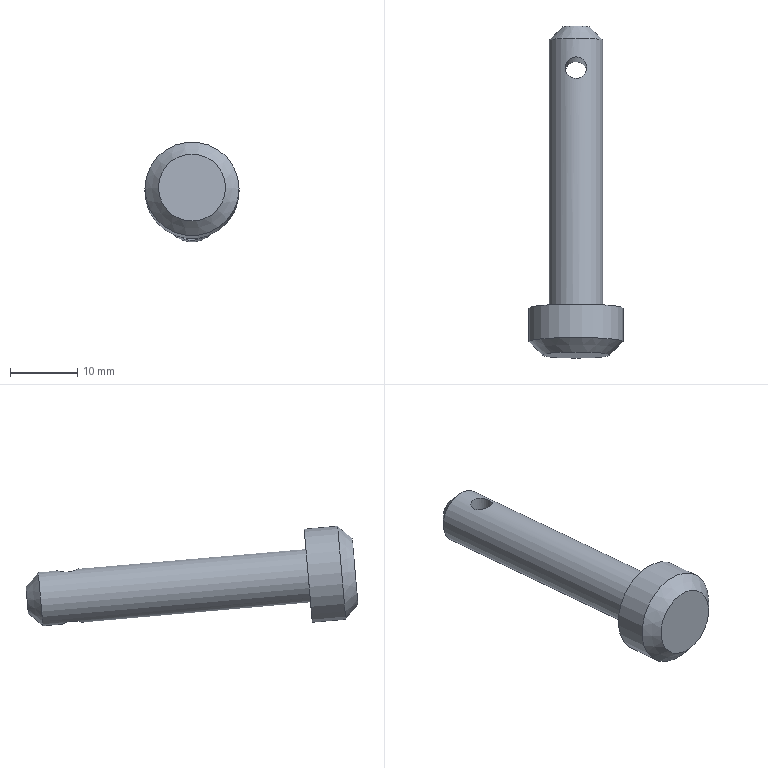Component | NX | PIN | 1 solid | 8 faces | box 14 x 49.42 x 14.88 mm | volume 3004 mm3 | cylinder 3 | plane 3 | cone 2 | commonest cylinder face diameters 8 x1 14 x1 3.2 x1
STEP:
#1=CARTESIAN_POINT('',(0.,0.,0.));
#2=DIRECTION('',(0.,0.,1.));
#3=DIRECTION('',(1.,0.,0.));
#4=AXIS2_PLACEMENT_3D('',#1,#2,#3);
#5=CARTESIAN_POINT('',(279.941,470.083,-25.853));
#6=VERTEX_POINT('',#5);
#7=CARTESIAN_POINT('',(275.941,470.083,-25.853));
#8=DIRECTION('',(0.,-0.9962,0.08716));
#9=DIRECTION('',(1.,0.,0.));
#10=AXIS2_PLACEMENT_3D('',#7,#8,#9);
#11=CIRCLE('',#10,4.);
#12=CARTESIAN_POINT('',(275.941,430.235,-22.367));
#13=DIRECTION('',(0.,0.9962,-0.08716));
#14=DIRECTION('',(-1.,0.,0.));
#15=AXIS2_PLACEMENT_3D('',#12,#13,#14);
#16=CYLINDRICAL_SURFACE('',#15,4.);
#17=CARTESIAN_POINT('',(9.425,40.));
#18=DIRECTION('',(-1.,0.));
#19=VECTOR('',#18,1.);
#20=LINE('',#17,#19);
#21=(GEOMETRIC_REPRESENTATION_CONTEXT(2)PARAMETRIC_REPRESENTATION_CONTEXT()REPRESENTATION_CONTEXT('',''));
#22=DEFINITIONAL_REPRESENTATION('',(#20),#21);
#23=PCURVE('',#16,#22);
#24=CARTESIAN_POINT('',(275.941,470.083,-25.853));
#25=DIRECTION('',(0.,-0.9962,0.08716));
#26=DIRECTION('',(1.,-0.,-0.));
#27=AXIS2_PLACEMENT_3D('',#24,#25,#26);
#28=CONICAL_SURFACE('',#27,4.,0.7854);
#29=CARTESIAN_POINT('',(0.,0.));
#30=DIRECTION('',(1.,0.));
#31=VECTOR('',#30,1.);
#32=LINE('',#29,#31);
#33=(GEOMETRIC_REPRESENTATION_CONTEXT(2)PARAMETRIC_REPRESENTATION_CONTEXT()REPRESENTATION_CONTEXT('',''));
#34=DEFINITIONAL_REPRESENTATION('',(#32),#33);
#35=PCURVE('',#28,#34);
#36=SURFACE_CURVE('',#11,(#23,#35),.PCURVE_S1.);
#37=EDGE_CURVE('',#6,#6,#36,.T.);
#38=ORIENTED_EDGE('',*,*,#37,.T.);
#39=CARTESIAN_POINT('',(279.941,430.235,-22.367));
#40=VERTEX_POINT('',#39);
#41=CARTESIAN_POINT('',(279.941,430.235,-22.367));
#42=CARTESIAN_POINT('',(279.941,470.083,-25.853));
#43=B_SPLINE_CURVE_WITH_KNOTS('',1,(#41,#42),.UNSPECIFIED.,.F.,.F.,(2,2),(0.,40.),.PIECEWISE_BEZIER_KNOTS.);
#44=CARTESIAN_POINT('',(3.142,0.));
#45=DIRECTION('',(0.,1.));
#46=VECTOR('',#45,1.);
#47=LINE('',#44,#46);
#48=(GEOMETRIC_REPRESENTATION_CONTEXT(2)PARAMETRIC_REPRESENTATION_CONTEXT()REPRESENTATION_CONTEXT('',''));
#49=DEFINITIONAL_REPRESENTATION('',(#47),#48);
#50=PCURVE('',#16,#49);
#51=CARTESIAN_POINT('',(9.425,0.));
#52=DIRECTION('',(0.,1.));
#53=VECTOR('',#52,1.);
#54=LINE('',#51,#53);
#55=(GEOMETRIC_REPRESENTATION_CONTEXT(2)PARAMETRIC_REPRESENTATION_CONTEXT()REPRESENTATION_CONTEXT('',''));
#56=DEFINITIONAL_REPRESENTATION('',(#54),#55);
#57=PCURVE('',#16,#56);
#58=SEAM_CURVE('',#43,(#50,#57),.PCURVE_S1.);
#59=EDGE_CURVE('',#40,#6,#58,.T.);
#60=ORIENTED_EDGE('',*,*,#59,.F.);
#61=CARTESIAN_POINT('',(275.941,430.235,-22.367));
#62=DIRECTION('',(0.,-0.9962,0.08716));
#63=DIRECTION('',(1.,0.,0.));
#64=AXIS2_PLACEMENT_3D('',#61,#62,#63);
#65=CIRCLE('',#64,4.);
#66=CARTESIAN_POINT('',(9.425,0.));
#67=DIRECTION('',(-1.,0.));
#68=VECTOR('',#67,1.);
#69=LINE('',#66,#68);
#70=(GEOMETRIC_REPRESENTATION_CONTEXT(2)PARAMETRIC_REPRESENTATION_CONTEXT()REPRESENTATION_CONTEXT('',''));
#71=DEFINITIONAL_REPRESENTATION('',(#69),#70);
#72=PCURVE('',#16,#71);
#73=CARTESIAN_POINT('',(275.941,430.235,-22.367));
#74=DIRECTION('',(0.,-0.9962,0.08716));
#75=DIRECTION('',(1.,0.,0.));
#76=AXIS2_PLACEMENT_3D('',#73,#74,#75);
#77=PLANE('',#76);
#78=CARTESIAN_POINT('',(0.,0.));
#79=DIRECTION('',(1.,0.));
#80=AXIS2_PLACEMENT_2D('',#78,#79);
#81=CIRCLE('',#80,4.);
#82=(GEOMETRIC_REPRESENTATION_CONTEXT(2)PARAMETRIC_REPRESENTATION_CONTEXT()REPRESENTATION_CONTEXT('',''));
#83=DEFINITIONAL_REPRESENTATION('',(#81),#82);
#84=PCURVE('',#77,#83);
#85=SURFACE_CURVE('',#65,(#72,#84),.PCURVE_S1.);
#86=EDGE_CURVE('',#40,#40,#85,.T.);
#87=ORIENTED_EDGE('',*,*,#86,.F.);
#88=ORIENTED_EDGE('',*,*,#59,.T.);
#89=EDGE_LOOP('',(#38,#60,#87,#88));
#90=FACE_BOUND('',#89,.T.);
#91=CARTESIAN_POINT('',(275.941,464.455,-21.345));
#92=VERTEX_POINT('',#91);
#93=CARTESIAN_POINT('',(275.941,464.455,-21.345));
#94=CARTESIAN_POINT('',(276.113,464.455,-21.345));
#95=CARTESIAN_POINT('',(276.287,464.482,-21.359));
#96=CARTESIAN_POINT('',(276.448,464.534,-21.384));
#97=CARTESIAN_POINT('',(276.609,464.586,-21.41));
#98=CARTESIAN_POINT('',(276.763,464.663,-21.446));
#99=CARTESIAN_POINT('',(276.897,464.761,-21.488));
#100=CARTESIAN_POINT('',(277.038,464.862,-21.532));
#101=CARTESIAN_POINT('',(277.162,464.987,-21.582));
#102=CARTESIAN_POINT('',(277.261,465.128,-21.629));
#103=CARTESIAN_POINT('',(277.364,465.275,-21.678));
#104=CARTESIAN_POINT('',(277.443,465.444,-21.725));
#105=CARTESIAN_POINT('',(277.49,465.621,-21.76));
#106=CARTESIAN_POINT('',(277.534,465.79,-21.794));
#107=CARTESIAN_POINT('',(277.55,465.972,-21.817));
#108=CARTESIAN_POINT('',(277.536,466.149,-21.826));
#109=CARTESIAN_POINT('',(277.522,466.314,-21.835));
#110=CARTESIAN_POINT('',(277.483,466.479,-21.832));
#111=CARTESIAN_POINT('',(277.42,466.632,-21.82));
#112=CARTESIAN_POINT('',(277.356,466.788,-21.808));
#113=CARTESIAN_POINT('',(277.268,466.935,-21.788));
#114=CARTESIAN_POINT('',(277.16,467.064,-21.764));
#115=CARTESIAN_POINT('',(277.045,467.203,-21.739));
#116=CARTESIAN_POINT('',(276.905,467.323,-21.711));
#117=CARTESIAN_POINT('',(276.75,467.417,-21.687));
#118=CARTESIAN_POINT('',(276.592,467.511,-21.663));
#119=CARTESIAN_POINT('',(276.415,467.58,-21.642));
#120=CARTESIAN_POINT('',(276.233,467.615,-21.632));
#121=CARTESIAN_POINT('',(276.061,467.648,-21.622));
#122=CARTESIAN_POINT('',(275.882,467.651,-21.621));
#123=CARTESIAN_POINT('',(275.709,467.625,-21.629));
#124=CARTESIAN_POINT('',(275.544,467.6,-21.637));
#125=CARTESIAN_POINT('',(275.382,467.548,-21.652));
#126=CARTESIAN_POINT('',(275.234,467.473,-21.672));
#127=CARTESIAN_POINT('',(275.082,467.396,-21.693));
#128=CARTESIAN_POINT('',(274.941,467.293,-21.719));
#129=CARTESIAN_POINT('',(274.821,467.173,-21.743));
#130=CARTESIAN_POINT('',(274.693,467.044,-21.77));
#131=CARTESIAN_POINT('',(274.585,466.892,-21.795));
#132=CARTESIAN_POINT('',(274.505,466.728,-21.812));
#133=CARTESIAN_POINT('',(274.425,466.562,-21.828));
#134=CARTESIAN_POINT('',(274.371,466.379,-21.836));
#135=CARTESIAN_POINT('',(274.351,466.195,-21.828));
#136=CARTESIAN_POINT('',(274.332,466.025,-21.822));
#137=CARTESIAN_POINT('',(274.341,465.849,-21.802));
#138=CARTESIAN_POINT('',(274.377,465.684,-21.772));
#139=CARTESIAN_POINT('',(274.412,465.525,-21.744));
#140=CARTESIAN_POINT('',(274.472,465.372,-21.705));
#141=CARTESIAN_POINT('',(274.553,465.235,-21.663));
#142=CARTESIAN_POINT('',(274.638,465.089,-21.618));
#143=CARTESIAN_POINT('',(274.748,464.957,-21.569));
#144=CARTESIAN_POINT('',(274.876,464.847,-21.524));
#145=CARTESIAN_POINT('',(275.011,464.729,-21.476));
#146=CARTESIAN_POINT('',(275.171,464.633,-21.432));
#147=CARTESIAN_POINT('',(275.341,464.567,-21.4));
#148=CARTESIAN_POINT('',(275.508,464.502,-21.369));
#149=CARTESIAN_POINT('',(275.691,464.464,-21.349));
#150=CARTESIAN_POINT('',(275.873,464.456,-21.346));
#151=CARTESIAN_POINT('',(275.896,464.455,-21.345));
#152=CARTESIAN_POINT('',(275.918,464.455,-21.345));
#153=CARTESIAN_POINT('',(275.941,464.455,-21.345));
#154=B_SPLINE_CURVE_WITH_KNOTS('',3,(#93,#94,#95,#96,#97,#98,#99,#100,#101,#102,#103,#104,#105,#106,#107,#108,#109,#110,#111,#112,#113,#114,#115,#116,#117,#118,#119,#120,#121,#122,#123,#124,#125,#126,#127,#128,#129,#130,#131,#132,#133,#134,#135,#136,#137,#138,#139,#140,#141,#142,#143,#144,#145,#146,#147,#148,#149,#150,#151,#152,#153),.UNSPECIFIED.,.T.,.F.,(1,3,3,3,3,3,3,3,3,3,3,3,3,3,3,3,3,3,3,3,3,3,1),(-0.006652,0.,0.05091,0.1017,0.1546,0.2101,0.2629,0.312,0.3621,0.4161,0.4713,0.5231,0.5725,0.6234,0.6778,0.7328,0.7837,0.8325,0.8842,0.9393,0.9933,1.,1.051),.UNSPECIFIED.);
#155=CARTESIAN_POINT('',(7.854,34.));
#156=CARTESIAN_POINT('',(7.864,34.));
#157=CARTESIAN_POINT('',(7.883,34.003));
#158=CARTESIAN_POINT('',(7.912,34.015));
#159=CARTESIAN_POINT('',(7.94,34.036));
#160=CARTESIAN_POINT('',(7.968,34.065));
#161=CARTESIAN_POINT('',(7.995,34.101));
#162=CARTESIAN_POINT('',(8.022,34.145));
#163=CARTESIAN_POINT('',(8.048,34.197));
#164=CARTESIAN_POINT('',(8.073,34.255));
#165=CARTESIAN_POINT('',(8.097,34.32));
#166=CARTESIAN_POINT('',(8.119,34.391));
#167=CARTESIAN_POINT('',(8.141,34.468));
#168=CARTESIAN_POINT('',(8.161,34.551));
#169=CARTESIAN_POINT('',(8.18,34.639));
#170=CARTESIAN_POINT('',(8.197,34.732));
#171=CARTESIAN_POINT('',(8.212,34.829));
#172=CARTESIAN_POINT('',(8.226,34.931));
#173=CARTESIAN_POINT('',(8.238,35.036));
#174=CARTESIAN_POINT('',(8.248,35.145));
#175=CARTESIAN_POINT('',(8.256,35.255));
#176=CARTESIAN_POINT('',(8.261,35.369));
#177=CARTESIAN_POINT('',(8.265,35.484));
#178=CARTESIAN_POINT('',(8.266,35.599));
#179=CARTESIAN_POINT('',(8.265,35.714));
#180=CARTESIAN_POINT('',(8.261,35.829));
#181=CARTESIAN_POINT('',(8.256,35.942));
#182=CARTESIAN_POINT('',(8.248,36.054));
#183=CARTESIAN_POINT('',(8.238,36.163));
#184=CARTESIAN_POINT('',(8.226,36.268));
#185=CARTESIAN_POINT('',(8.213,36.37));
#186=CARTESIAN_POINT('',(8.197,36.467));
#187=CARTESIAN_POINT('',(8.18,36.561));
#188=CARTESIAN_POINT('',(8.161,36.649));
#189=CARTESIAN_POINT('',(8.141,36.731));
#190=CARTESIAN_POINT('',(8.12,36.809));
#191=CARTESIAN_POINT('',(8.097,36.88));
#192=CARTESIAN_POINT('',(8.073,36.945));
#193=CARTESIAN_POINT('',(8.048,37.003));
#194=CARTESIAN_POINT('',(8.022,37.054));
#195=CARTESIAN_POINT('',(7.996,37.098));
#196=CARTESIAN_POINT('',(7.968,37.135));
#197=CARTESIAN_POINT('',(7.94,37.164));
#198=CARTESIAN_POINT('',(7.912,37.184));
#199=CARTESIAN_POINT('',(7.883,37.197));
#200=CARTESIAN_POINT('',(7.854,37.201));
#201=CARTESIAN_POINT('',(7.825,37.197));
#202=CARTESIAN_POINT('',(7.797,37.185));
#203=CARTESIAN_POINT('',(7.768,37.164));
#204=CARTESIAN_POINT('',(7.74,37.136));
#205=CARTESIAN_POINT('',(7.713,37.099));
#206=CARTESIAN_POINT('',(7.686,37.055));
#207=CARTESIAN_POINT('',(7.66,37.004));
#208=CARTESIAN_POINT('',(7.635,36.946));
#209=CARTESIAN_POINT('',(7.611,36.881));
#210=CARTESIAN_POINT('',(7.589,36.809));
#211=CARTESIAN_POINT('',(7.567,36.733));
#212=CARTESIAN_POINT('',(7.547,36.65));
#213=CARTESIAN_POINT('',(7.528,36.562));
#214=CARTESIAN_POINT('',(7.511,36.469));
#215=CARTESIAN_POINT('',(7.495,36.371));
#216=CARTESIAN_POINT('',(7.482,36.27));
#217=CARTESIAN_POINT('',(7.47,36.165));
#218=CARTESIAN_POINT('',(7.46,36.056));
#219=CARTESIAN_POINT('',(7.452,35.944));
#220=CARTESIAN_POINT('',(7.447,35.831));
#221=CARTESIAN_POINT('',(7.443,35.717));
#222=CARTESIAN_POINT('',(7.442,35.602));
#223=CARTESIAN_POINT('',(7.443,35.486));
#224=CARTESIAN_POINT('',(7.447,35.371));
#225=CARTESIAN_POINT('',(7.452,35.258));
#226=CARTESIAN_POINT('',(7.46,35.147));
#227=CARTESIAN_POINT('',(7.47,35.038));
#228=CARTESIAN_POINT('',(7.482,34.932));
#229=CARTESIAN_POINT('',(7.495,34.83));
#230=CARTESIAN_POINT('',(7.511,34.733));
#231=CARTESIAN_POINT('',(7.528,34.639));
#232=CARTESIAN_POINT('',(7.547,34.551));
#233=CARTESIAN_POINT('',(7.567,34.468));
#234=CARTESIAN_POINT('',(7.588,34.391));
#235=CARTESIAN_POINT('',(7.611,34.32));
#236=CARTESIAN_POINT('',(7.635,34.255));
#237=CARTESIAN_POINT('',(7.66,34.197));
#238=CARTESIAN_POINT('',(7.686,34.145));
#239=CARTESIAN_POINT('',(7.712,34.101));
#240=CARTESIAN_POINT('',(7.74,34.065));
#241=CARTESIAN_POINT('',(7.768,34.036));
#242=CARTESIAN_POINT('',(7.796,34.015));
#243=CARTESIAN_POINT('',(7.825,34.003));
#244=CARTESIAN_POINT('',(7.844,34.));
#245=CARTESIAN_POINT('',(7.854,34.));
#246=B_SPLINE_CURVE_WITH_KNOTS('',3,(#155,#156,#157,#158,#159,#160,#161,#162,#163,#164,#165,#166,#167,#168,#169,#170,#171,#172,#173,#174,#175,#176,#177,#178,#179,#180,#181,#182,#183,#184,#185,#186,#187,#188,#189,#190,#191,#192,#193,#194,#195,#196,#197,#198,#199,#200,#201,#202,#203,#204,#205,#206,#207,#208,#209,#210,#211,#212,#213,#214,#215,#216,#217,#218,#219,#220,#221,#222,#223,#224,#225,#226,#227,#228,#229,#230,#231,#232,#233,#234,#235,#236,#237,#238,#239,#240,#241,#242,#243,#244,#245),.UNSPECIFIED.,.T.,.F.,(4,1,1,1,1,1,1,1,1,1,1,1,1,1,1,1,1,1,1,1,1,1,1,1,1,1,1,1,1,1,1,1,1,1,1,1,1,1,1,1,1,1,1,1,1,1,1,1,1,1,1,1,1,1,1,1,1,1,1,1,1,1,1,1,1,1,1,1,1,1,1,1,1,1,1,1,1,1,1,1,1,1,1,1,1,1,1,1,4),(0.,0.01136,0.02273,0.03409,0.04545,0.05682,0.06818,0.07955,0.09091,0.1023,0.1136,0.125,0.1364,0.1477,0.1591,0.1705,0.1818,0.1932,0.2045,0.2159,0.2273,0.2386,0.25,0.2614,0.2727,0.2841,0.2955,0.3068,0.3182,0.3295,0.3409,0.3523,0.3636,0.375,0.3864,0.3977,0.4091,0.4205,0.4318,0.4432,0.4545,0.4659,0.4773,0.4886,0.5,0.5114,0.5227,0.5341,0.5455,0.5568,0.5682,0.5795,0.5909,0.6023,0.6136,0.625,0.6364,0.6477,0.6591,0.6705,0.6818,0.6932,0.7045,0.7159,0.7273,0.7386,0.75,0.7614,0.7727,0.7841,0.7955,0.8068,0.8182,0.8295,0.8409,0.8523,0.8636,0.875,0.8864,0.8977,0.9091,0.9205,0.9318,0.9432,0.9545,0.9659,0.9773,0.9886,1.),.QUASI_UNIFORM_KNOTS.);
#247=(GEOMETRIC_REPRESENTATION_CONTEXT(2)PARAMETRIC_REPRESENTATION_CONTEXT()REPRESENTATION_CONTEXT('',''));
#248=DEFINITIONAL_REPRESENTATION('',(#246),#247);
#249=PCURVE('',#16,#248);
#250=CARTESIAN_POINT('',(275.941,465.09,-32.443));
#251=DIRECTION('',(0.,0.08716,0.9962));
#252=DIRECTION('',(0.,-0.9962,0.08716));
#253=AXIS2_PLACEMENT_3D('',#250,#251,#252);
#254=CYLINDRICAL_SURFACE('',#253,1.6);
#255=CARTESIAN_POINT('',(0.,11.));
#256=CARTESIAN_POINT('',(0.02393,11.));
#257=CARTESIAN_POINT('',(0.07194,10.999));
#258=CARTESIAN_POINT('',(0.1442,10.994));
#259=CARTESIAN_POINT('',(0.2163,10.986));
#260=CARTESIAN_POINT('',(0.2882,10.975));
#261=CARTESIAN_POINT('',(0.3595,10.961));
#262=CARTESIAN_POINT('',(0.431,10.944));
#263=CARTESIAN_POINT('',(0.5024,10.925));
#264=CARTESIAN_POINT('',(0.5736,10.905));
#265=CARTESIAN_POINT('',(0.6443,10.883));
#266=CARTESIAN_POINT('',(0.7148,10.86));
#267=CARTESIAN_POINT('',(0.7857,10.837));
#268=CARTESIAN_POINT('',(0.8565,10.813));
#269=CARTESIAN_POINT('',(0.9272,10.79));
#270=CARTESIAN_POINT('',(0.9976,10.767));
#271=CARTESIAN_POINT('',(1.068,10.746));
#272=CARTESIAN_POINT('',(1.14,10.726));
#273=CARTESIAN_POINT('',(1.211,10.709));
#274=CARTESIAN_POINT('',(1.283,10.694));
#275=CARTESIAN_POINT('',(1.354,10.682));
#276=CARTESIAN_POINT('',(1.426,10.673));
#277=CARTESIAN_POINT('',(1.498,10.667));
#278=CARTESIAN_POINT('',(1.57,10.666));
#279=CARTESIAN_POINT('',(1.642,10.667));
#280=CARTESIAN_POINT('',(1.714,10.673));
#281=CARTESIAN_POINT('',(1.786,10.682));
#282=CARTESIAN_POINT('',(1.858,10.694));
#283=CARTESIAN_POINT('',(1.93,10.708));
#284=CARTESIAN_POINT('',(2.001,10.726));
#285=CARTESIAN_POINT('',(2.072,10.746));
#286=CARTESIAN_POINT('',(2.143,10.767));
#287=CARTESIAN_POINT('',(2.214,10.79));
#288=CARTESIAN_POINT('',(2.285,10.813));
#289=CARTESIAN_POINT('',(2.355,10.836));
#290=CARTESIAN_POINT('',(2.426,10.86));
#291=CARTESIAN_POINT('',(2.497,10.883));
#292=CARTESIAN_POINT('',(2.568,10.905));
#293=CARTESIAN_POINT('',(2.639,10.925));
#294=CARTESIAN_POINT('',(2.71,10.944));
#295=CARTESIAN_POINT('',(2.781,10.96));
#296=CARTESIAN_POINT('',(2.853,10.974));
#297=CARTESIAN_POINT('',(2.925,10.986));
#298=CARTESIAN_POINT('',(2.996,10.994));
#299=CARTESIAN_POINT('',(3.068,10.999));
#300=CARTESIAN_POINT('',(3.141,11.));
#301=CARTESIAN_POINT('',(3.213,10.999));
#302=CARTESIAN_POINT('',(3.285,10.994));
#303=CARTESIAN_POINT('',(3.357,10.986));
#304=CARTESIAN_POINT('',(3.429,10.975));
#305=CARTESIAN_POINT('',(3.501,10.961));
#306=CARTESIAN_POINT('',(3.572,10.944));
#307=CARTESIAN_POINT('',(3.643,10.926));
#308=CARTESIAN_POINT('',(3.714,10.905));
#309=CARTESIAN_POINT('',(3.785,10.883));
#310=CARTESIAN_POINT('',(3.856,10.86));
#311=CARTESIAN_POINT('',(3.927,10.837));
#312=CARTESIAN_POINT('',(3.997,10.813));
#313=CARTESIAN_POINT('',(4.068,10.79));
#314=CARTESIAN_POINT('',(4.139,10.767));
#315=CARTESIAN_POINT('',(4.21,10.746));
#316=CARTESIAN_POINT('',(4.281,10.726));
#317=CARTESIAN_POINT('',(4.352,10.709));
#318=CARTESIAN_POINT('',(4.424,10.694));
#319=CARTESIAN_POINT('',(4.496,10.682));
#320=CARTESIAN_POINT('',(4.567,10.673));
#321=CARTESIAN_POINT('',(4.639,10.667));
#322=CARTESIAN_POINT('',(4.711,10.666));
#323=CARTESIAN_POINT('',(4.784,10.667));
#324=CARTESIAN_POINT('',(4.856,10.673));
#325=CARTESIAN_POINT('',(4.928,10.681));
#326=CARTESIAN_POINT('',(4.999,10.693));
#327=CARTESIAN_POINT('',(5.071,10.709));
#328=CARTESIAN_POINT('',(5.143,10.726));
#329=CARTESIAN_POINT('',(5.214,10.746));
#330=CARTESIAN_POINT('',(5.285,10.767));
#331=CARTESIAN_POINT('',(5.356,10.79));
#332=CARTESIAN_POINT('',(5.427,10.813));
#333=CARTESIAN_POINT('',(5.498,10.837));
#334=CARTESIAN_POINT('',(5.568,10.86));
#335=CARTESIAN_POINT('',(5.639,10.883));
#336=CARTESIAN_POINT('',(5.71,10.905));
#337=CARTESIAN_POINT('',(5.781,10.925));
#338=CARTESIAN_POINT('',(5.852,10.944));
#339=CARTESIAN_POINT('',(5.923,10.96));
#340=CARTESIAN_POINT('',(5.995,10.974));
#341=CARTESIAN_POINT('',(6.067,10.986));
#342=CARTESIAN_POINT('',(6.139,10.994));
#343=CARTESIAN_POINT('',(6.211,10.999));
#344=CARTESIAN_POINT('',(6.259,11.));
#345=CARTESIAN_POINT('',(6.283,11.));
#346=B_SPLINE_CURVE_WITH_KNOTS('',3,(#255,#256,#257,#258,#259,#260,#261,#262,#263,#264,#265,#266,#267,#268,#269,#270,#271,#272,#273,#274,#275,#276,#277,#278,#279,#280,#281,#282,#283,#284,#285,#286,#287,#288,#289,#290,#291,#292,#293,#294,#295,#296,#297,#298,#299,#300,#301,#302,#303,#304,#305,#306,#307,#308,#309,#310,#311,#312,#313,#314,#315,#316,#317,#318,#319,#320,#321,#322,#323,#324,#325,#326,#327,#328,#329,#330,#331,#332,#333,#334,#335,#336,#337,#338,#339,#340,#341,#342,#343,#344,#345),.UNSPECIFIED.,.F.,.F.,(4,1,1,1,1,1,1,1,1,1,1,1,1,1,1,1,1,1,1,1,1,1,1,1,1,1,1,1,1,1,1,1,1,1,1,1,1,1,1,1,1,1,1,1,1,1,1,1,1,1,1,1,1,1,1,1,1,1,1,1,1,1,1,1,1,1,1,1,1,1,1,1,1,1,1,1,1,1,1,1,1,1,1,1,1,1,1,1,4),(0.,0.01136,0.02273,0.03409,0.04545,0.05682,0.06818,0.07955,0.09091,0.1023,0.1136,0.125,0.1364,0.1477,0.1591,0.1705,0.1818,0.1932,0.2045,0.2159,0.2273,0.2386,0.25,0.2614,0.2727,0.2841,0.2955,0.3068,0.3182,0.3295,0.3409,0.3523,0.3636,0.375,0.3864,0.3977,0.4091,0.4205,0.4318,0.4432,0.4545,0.4659,0.4773,0.4886,0.5,0.5114,0.5227,0.5341,0.5455,0.5568,0.5682,0.5795,0.5909,0.6023,0.6136,0.625,0.6364,0.6477,0.6591,0.6705,0.6818,0.6932,0.7045,0.7159,0.7273,0.7386,0.75,0.7614,0.7727,0.7841,0.7955,0.8068,0.8182,0.8295,0.8409,0.8523,0.8636,0.875,0.8864,0.8977,0.9091,0.9205,0.9318,0.9432,0.9545,0.9659,0.9773,0.9886,1.),.QUASI_UNIFORM_KNOTS.);
#347=(GEOMETRIC_REPRESENTATION_CONTEXT(2)PARAMETRIC_REPRESENTATION_CONTEXT()REPRESENTATION_CONTEXT('',''));
#348=DEFINITIONAL_REPRESENTATION('',(#346),#347);
#349=PCURVE('',#254,#348);
#350=SURFACE_CURVE('',#154,(#249,#349),.PCURVE_S1.);
#351=EDGE_CURVE('',#92,#92,#350,.T.);
#352=ORIENTED_EDGE('',*,*,#351,.F.);
#353=EDGE_LOOP('',(#352));
#354=FACE_BOUND('',#353,.T.);
#355=CARTESIAN_POINT('',(275.941,463.757,-29.315));
#356=VERTEX_POINT('',#355);
#357=CARTESIAN_POINT('',(275.941,463.757,-29.315));
#358=CARTESIAN_POINT('',(275.77,463.757,-29.315));
#359=CARTESIAN_POINT('',(275.596,463.787,-29.305));
#360=CARTESIAN_POINT('',(275.434,463.842,-29.29));
#361=CARTESIAN_POINT('',(275.273,463.898,-29.274));
#362=CARTESIAN_POINT('',(275.12,463.981,-29.251));
#363=CARTESIAN_POINT('',(274.985,464.084,-29.227));
#364=CARTESIAN_POINT('',(274.844,464.191,-29.201));
#365=CARTESIAN_POINT('',(274.72,464.323,-29.174));
#366=CARTESIAN_POINT('',(274.621,464.47,-29.152));
#367=CARTESIAN_POINT('',(274.518,464.623,-29.129));
#368=CARTESIAN_POINT('',(274.439,464.798,-29.112));
#369=CARTESIAN_POINT('',(274.392,464.979,-29.108));
#370=CARTESIAN_POINT('',(274.348,465.151,-29.105));
#371=CARTESIAN_POINT('',(274.332,465.334,-29.113));
#372=CARTESIAN_POINT('',(274.346,465.509,-29.135));
#373=CARTESIAN_POINT('',(274.36,465.673,-29.155));
#374=CARTESIAN_POINT('',(274.4,465.836,-29.187));
#375=CARTESIAN_POINT('',(274.462,465.984,-29.225));
#376=CARTESIAN_POINT('',(274.526,466.136,-29.264));
#377=CARTESIAN_POINT('',(274.615,466.277,-29.31));
#378=CARTESIAN_POINT('',(274.722,466.4,-29.355));
#379=CARTESIAN_POINT('',(274.837,466.532,-29.403));
#380=CARTESIAN_POINT('',(274.977,466.646,-29.452));
#381=CARTESIAN_POINT('',(275.132,466.734,-29.492));
#382=CARTESIAN_POINT('',(275.29,466.823,-29.532));
#383=CARTESIAN_POINT('',(275.468,466.887,-29.564));
#384=CARTESIAN_POINT('',(275.65,466.919,-29.581));
#385=CARTESIAN_POINT('',(275.821,466.95,-29.596));
#386=CARTESIAN_POINT('',(276.001,466.953,-29.597));
#387=CARTESIAN_POINT('',(276.173,466.929,-29.585));
#388=CARTESIAN_POINT('',(276.338,466.906,-29.574));
#389=CARTESIAN_POINT('',(276.5,466.857,-29.549));
#390=CARTESIAN_POINT('',(276.648,466.787,-29.516));
#391=CARTESIAN_POINT('',(276.8,466.714,-29.483));
#392=CARTESIAN_POINT('',(276.941,466.618,-29.439));
#393=CARTESIAN_POINT('',(277.061,466.503,-29.394));
#394=CARTESIAN_POINT('',(277.189,466.381,-29.346));
#395=CARTESIAN_POINT('',(277.298,466.236,-29.294));
#396=CARTESIAN_POINT('',(277.377,466.077,-29.25));
#397=CARTESIAN_POINT('',(277.458,465.917,-29.205));
#398=CARTESIAN_POINT('',(277.511,465.737,-29.166));
#399=CARTESIAN_POINT('',(277.531,465.555,-29.141));
#400=CARTESIAN_POINT('',(277.55,465.386,-29.118));
#401=CARTESIAN_POINT('',(277.541,465.21,-29.107));
#402=CARTESIAN_POINT('',(277.505,465.042,-29.107));
#403=CARTESIAN_POINT('',(277.47,464.881,-29.108));
#404=CARTESIAN_POINT('',(277.41,464.723,-29.12));
#405=CARTESIAN_POINT('',(277.329,464.581,-29.137));
#406=CARTESIAN_POINT('',(277.244,464.43,-29.155));
#407=CARTESIAN_POINT('',(277.134,464.291,-29.181));
#408=CARTESIAN_POINT('',(277.006,464.175,-29.206));
#409=CARTESIAN_POINT('',(276.871,464.051,-29.233));
#410=CARTESIAN_POINT('',(276.711,463.949,-29.26));
#411=CARTESIAN_POINT('',(276.541,463.878,-29.28));
#412=CARTESIAN_POINT('',(276.374,463.808,-29.299));
#413=CARTESIAN_POINT('',(276.191,463.767,-29.312));
#414=CARTESIAN_POINT('',(276.009,463.759,-29.314));
#415=CARTESIAN_POINT('',(275.987,463.758,-29.314));
#416=CARTESIAN_POINT('',(275.964,463.757,-29.315));
#417=CARTESIAN_POINT('',(275.941,463.757,-29.315));
#418=B_SPLINE_CURVE_WITH_KNOTS('',3,(#357,#358,#359,#360,#361,#362,#363,#364,#365,#366,#367,#368,#369,#370,#371,#372,#373,#374,#375,#376,#377,#378,#379,#380,#381,#382,#383,#384,#385,#386,#387,#388,#389,#390,#391,#392,#393,#394,#395,#396,#397,#398,#399,#400,#401,#402,#403,#404,#405,#406,#407,#408,#409,#410,#411,#412,#413,#414,#415,#416,#417),.UNSPECIFIED.,.T.,.F.,(1,3,3,3,3,3,3,3,3,3,3,3,3,3,3,3,3,3,3,3,3,3,1),(-0.006652,0.,0.05091,0.1017,0.1546,0.2101,0.2629,0.312,0.3621,0.4161,0.4713,0.5231,0.5725,0.6234,0.6778,0.7328,0.7837,0.8325,0.8842,0.9393,0.9933,1.,1.051),.UNSPECIFIED.);
#419=CARTESIAN_POINT('',(4.712,34.));
#420=CARTESIAN_POINT('',(4.722,34.));
#421=CARTESIAN_POINT('',(4.741,34.003));
#422=CARTESIAN_POINT('',(4.77,34.015));
#423=CARTESIAN_POINT('',(4.798,34.036));
#424=CARTESIAN_POINT('',(4.826,34.065));
#425=CARTESIAN_POINT('',(4.854,34.101));
#426=CARTESIAN_POINT('',(4.88,34.145));
#427=CARTESIAN_POINT('',(4.906,34.197));
#428=CARTESIAN_POINT('',(4.931,34.255));
#429=CARTESIAN_POINT('',(4.955,34.32));
#430=CARTESIAN_POINT('',(4.978,34.391));
#431=CARTESIAN_POINT('',(4.999,34.468));
#432=CARTESIAN_POINT('',(5.02,34.551));
#433=CARTESIAN_POINT('',(5.038,34.639));
#434=CARTESIAN_POINT('',(5.055,34.732));
#435=CARTESIAN_POINT('',(5.071,34.829));
#436=CARTESIAN_POINT('',(5.085,34.931));
#437=CARTESIAN_POINT('',(5.096,35.036));
#438=CARTESIAN_POINT('',(5.106,35.145));
#439=CARTESIAN_POINT('',(5.114,35.255));
#440=CARTESIAN_POINT('',(5.12,35.369));
#441=CARTESIAN_POINT('',(5.123,35.484));
#442=CARTESIAN_POINT('',(5.124,35.599));
#443=CARTESIAN_POINT('',(5.123,35.714));
#444=CARTESIAN_POINT('',(5.12,35.829));
#445=CARTESIAN_POINT('',(5.114,35.942));
#446=CARTESIAN_POINT('',(5.106,36.054));
#447=CARTESIAN_POINT('',(5.097,36.163));
#448=CARTESIAN_POINT('',(5.085,36.268));
#449=CARTESIAN_POINT('',(5.071,36.37));
#450=CARTESIAN_POINT('',(5.056,36.467));
#451=CARTESIAN_POINT('',(5.038,36.561));
#452=CARTESIAN_POINT('',(5.02,36.649));
#453=CARTESIAN_POINT('',(5.,36.731));
#454=CARTESIAN_POINT('',(4.978,36.809));
#455=CARTESIAN_POINT('',(4.955,36.88));
#456=CARTESIAN_POINT('',(4.931,36.945));
#457=CARTESIAN_POINT('',(4.907,37.003));
#458=CARTESIAN_POINT('',(4.881,37.054));
#459=CARTESIAN_POINT('',(4.854,37.098));
#460=CARTESIAN_POINT('',(4.827,37.135));
#461=CARTESIAN_POINT('',(4.799,37.164));
#462=CARTESIAN_POINT('',(4.77,37.184));
#463=CARTESIAN_POINT('',(4.742,37.197));
#464=CARTESIAN_POINT('',(4.713,37.201));
#465=CARTESIAN_POINT('',(4.684,37.197));
#466=CARTESIAN_POINT('',(4.655,37.185));
#467=CARTESIAN_POINT('',(4.627,37.164));
#468=CARTESIAN_POINT('',(4.599,37.136));
#469=CARTESIAN_POINT('',(4.571,37.099));
#470=CARTESIAN_POINT('',(4.545,37.055));
#471=CARTESIAN_POINT('',(4.519,37.004));
#472=CARTESIAN_POINT('',(4.494,36.946));
#473=CARTESIAN_POINT('',(4.47,36.881));
#474=CARTESIAN_POINT('',(4.447,36.809));
#475=CARTESIAN_POINT('',(4.425,36.733));
#476=CARTESIAN_POINT('',(4.405,36.65));
#477=CARTESIAN_POINT('',(4.387,36.562));
#478=CARTESIAN_POINT('',(4.369,36.469));
#479=CARTESIAN_POINT('',(4.354,36.371));
#480=CARTESIAN_POINT('',(4.34,36.27));
#481=CARTESIAN_POINT('',(4.328,36.165));
#482=CARTESIAN_POINT('',(4.319,36.056));
#483=CARTESIAN_POINT('',(4.311,35.944));
#484=CARTESIAN_POINT('',(4.305,35.831));
#485=CARTESIAN_POINT('',(4.302,35.717));
#486=CARTESIAN_POINT('',(4.301,35.602));
#487=CARTESIAN_POINT('',(4.302,35.486));
#488=CARTESIAN_POINT('',(4.305,35.371));
#489=CARTESIAN_POINT('',(4.311,35.258));
#490=CARTESIAN_POINT('',(4.318,35.147));
#491=CARTESIAN_POINT('',(4.328,35.038));
#492=CARTESIAN_POINT('',(4.34,34.932));
#493=CARTESIAN_POINT('',(4.354,34.83));
#494=CARTESIAN_POINT('',(4.369,34.733));
#495=CARTESIAN_POINT('',(4.386,34.639));
#496=CARTESIAN_POINT('',(4.405,34.551));
#497=CARTESIAN_POINT('',(4.425,34.468));
#498=CARTESIAN_POINT('',(4.447,34.391));
#499=CARTESIAN_POINT('',(4.469,34.32));
#500=CARTESIAN_POINT('',(4.493,34.255));
#501=CARTESIAN_POINT('',(4.518,34.197));
#502=CARTESIAN_POINT('',(4.544,34.145));
#503=CARTESIAN_POINT('',(4.571,34.101));
#504=CARTESIAN_POINT('',(4.598,34.065));
#505=CARTESIAN_POINT('',(4.626,34.036));
#506=CARTESIAN_POINT('',(4.655,34.015));
#507=CARTESIAN_POINT('',(4.683,34.003));
#508=CARTESIAN_POINT('',(4.703,34.));
#509=CARTESIAN_POINT('',(4.712,34.));
#510=B_SPLINE_CURVE_WITH_KNOTS('',3,(#419,#420,#421,#422,#423,#424,#425,#426,#427,#428,#429,#430,#431,#432,#433,#434,#435,#436,#437,#438,#439,#440,#441,#442,#443,#444,#445,#446,#447,#448,#449,#450,#451,#452,#453,#454,#455,#456,#457,#458,#459,#460,#461,#462,#463,#464,#465,#466,#467,#468,#469,#470,#471,#472,#473,#474,#475,#476,#477,#478,#479,#480,#481,#482,#483,#484,#485,#486,#487,#488,#489,#490,#491,#492,#493,#494,#495,#496,#497,#498,#499,#500,#501,#502,#503,#504,#505,#506,#507,#508,#509),.UNSPECIFIED.,.T.,.F.,(4,1,1,1,1,1,1,1,1,1,1,1,1,1,1,1,1,1,1,1,1,1,1,1,1,1,1,1,1,1,1,1,1,1,1,1,1,1,1,1,1,1,1,1,1,1,1,1,1,1,1,1,1,1,1,1,1,1,1,1,1,1,1,1,1,1,1,1,1,1,1,1,1,1,1,1,1,1,1,1,1,1,1,1,1,1,1,1,4),(0.,0.01136,0.02273,0.03409,0.04545,0.05682,0.06818,0.07955,0.09091,0.1023,0.1136,0.125,0.1364,0.1477,0.1591,0.1705,0.1818,0.1932,0.2045,0.2159,0.2273,0.2386,0.25,0.2614,0.2727,0.2841,0.2955,0.3068,0.3182,0.3295,0.3409,0.3523,0.3636,0.375,0.3864,0.3977,0.4091,0.4205,0.4318,0.4432,0.4545,0.4659,0.4773,0.4886,0.5,0.5114,0.5227,0.5341,0.5455,0.5568,0.5682,0.5795,0.5909,0.6023,0.6136,0.625,0.6364,0.6477,0.6591,0.6705,0.6818,0.6932,0.7045,0.7159,0.7273,0.7386,0.75,0.7614,0.7727,0.7841,0.7955,0.8068,0.8182,0.8295,0.8409,0.8523,0.8636,0.875,0.8864,0.8977,0.9091,0.9205,0.9318,0.9432,0.9545,0.9659,0.9773,0.9886,1.),.QUASI_UNIFORM_KNOTS.);
#511=(GEOMETRIC_REPRESENTATION_CONTEXT(2)PARAMETRIC_REPRESENTATION_CONTEXT()REPRESENTATION_CONTEXT('',''));
#512=DEFINITIONAL_REPRESENTATION('',(#510),#511);
#513=PCURVE('',#16,#512);
#514=CARTESIAN_POINT('',(6.283,3.));
#515=CARTESIAN_POINT('',(6.259,3.));
#516=CARTESIAN_POINT('',(6.211,3.001));
#517=CARTESIAN_POINT('',(6.139,3.006));
#518=CARTESIAN_POINT('',(6.067,3.014));
#519=CARTESIAN_POINT('',(5.995,3.025));
#520=CARTESIAN_POINT('',(5.924,3.039));
#521=CARTESIAN_POINT('',(5.852,3.056));
#522=CARTESIAN_POINT('',(5.781,3.075));
#523=CARTESIAN_POINT('',(5.71,3.095));
#524=CARTESIAN_POINT('',(5.639,3.117));
#525=CARTESIAN_POINT('',(5.568,3.14));
#526=CARTESIAN_POINT('',(5.498,3.163));
#527=CARTESIAN_POINT('',(5.427,3.187));
#528=CARTESIAN_POINT('',(5.356,3.21));
#529=CARTESIAN_POINT('',(5.286,3.233));
#530=CARTESIAN_POINT('',(5.215,3.254));
#531=CARTESIAN_POINT('',(5.144,3.274));
#532=CARTESIAN_POINT('',(5.072,3.291));
#533=CARTESIAN_POINT('',(5.001,3.306));
#534=CARTESIAN_POINT('',(4.929,3.318));
#535=CARTESIAN_POINT('',(4.857,3.327));
#536=CARTESIAN_POINT('',(4.785,3.333));
#537=CARTESIAN_POINT('',(4.713,3.334));
#538=CARTESIAN_POINT('',(4.641,3.333));
#539=CARTESIAN_POINT('',(4.569,3.327));
#540=CARTESIAN_POINT('',(4.497,3.318));
#541=CARTESIAN_POINT('',(4.425,3.306));
#542=CARTESIAN_POINT('',(4.353,3.292));
#543=CARTESIAN_POINT('',(4.282,3.274));
#544=CARTESIAN_POINT('',(4.211,3.254));
#545=CARTESIAN_POINT('',(4.14,3.233));
#546=CARTESIAN_POINT('',(4.069,3.21));
#547=CARTESIAN_POINT('',(3.998,3.187));
#548=CARTESIAN_POINT('',(3.928,3.164));
#549=CARTESIAN_POINT('',(3.857,3.14));
#550=CARTESIAN_POINT('',(3.786,3.117));
#551=CARTESIAN_POINT('',(3.715,3.095));
#552=CARTESIAN_POINT('',(3.645,3.075));
#553=CARTESIAN_POINT('',(3.574,3.056));
#554=CARTESIAN_POINT('',(3.502,3.04));
#555=CARTESIAN_POINT('',(3.43,3.026));
#556=CARTESIAN_POINT('',(3.358,3.014));
#557=CARTESIAN_POINT('',(3.287,3.006));
#558=CARTESIAN_POINT('',(3.215,3.001));
#559=CARTESIAN_POINT('',(3.142,3.));
#560=CARTESIAN_POINT('',(3.07,3.001));
#561=CARTESIAN_POINT('',(2.998,3.006));
#562=CARTESIAN_POINT('',(2.926,3.014));
#563=CARTESIAN_POINT('',(2.854,3.025));
#564=CARTESIAN_POINT('',(2.783,3.039));
#565=CARTESIAN_POINT('',(2.711,3.056));
#566=CARTESIAN_POINT('',(2.64,3.074));
#567=CARTESIAN_POINT('',(2.569,3.095));
#568=CARTESIAN_POINT('',(2.498,3.117));
#569=CARTESIAN_POINT('',(2.427,3.14));
#570=CARTESIAN_POINT('',(2.356,3.163));
#571=CARTESIAN_POINT('',(2.286,3.187));
#572=CARTESIAN_POINT('',(2.215,3.21));
#573=CARTESIAN_POINT('',(2.144,3.233));
#574=CARTESIAN_POINT('',(2.073,3.254));
#575=CARTESIAN_POINT('',(2.002,3.274));
#576=CARTESIAN_POINT('',(1.931,3.291));
#577=CARTESIAN_POINT('',(1.859,3.306));
#578=CARTESIAN_POINT('',(1.788,3.318));
#579=CARTESIAN_POINT('',(1.716,3.327));
#580=CARTESIAN_POINT('',(1.644,3.333));
#581=CARTESIAN_POINT('',(1.572,3.334));
#582=CARTESIAN_POINT('',(1.499,3.333));
#583=CARTESIAN_POINT('',(1.427,3.327));
#584=CARTESIAN_POINT('',(1.355,3.319));
#585=CARTESIAN_POINT('',(1.284,3.307));
#586=CARTESIAN_POINT('',(1.212,3.291));
#587=CARTESIAN_POINT('',(1.14,3.274));
#588=CARTESIAN_POINT('',(1.069,3.254));
#589=CARTESIAN_POINT('',(0.9984,3.233));
#590=CARTESIAN_POINT('',(0.9274,3.21));
#591=CARTESIAN_POINT('',(0.8565,3.187));
#592=CARTESIAN_POINT('',(0.7857,3.163));
#593=CARTESIAN_POINT('',(0.7152,3.14));
#594=CARTESIAN_POINT('',(0.6446,3.117));
#595=CARTESIAN_POINT('',(0.5736,3.095));
#596=CARTESIAN_POINT('',(0.5024,3.075));
#597=CARTESIAN_POINT('',(0.4312,3.056));
#598=CARTESIAN_POINT('',(0.3601,3.04));
#599=CARTESIAN_POINT('',(0.2886,3.026));
#600=CARTESIAN_POINT('',(0.2166,3.014));
#601=CARTESIAN_POINT('',(0.1444,3.006));
#602=CARTESIAN_POINT('',(0.07254,3.001));
#603=CARTESIAN_POINT('',(0.02429,3.));
#604=CARTESIAN_POINT('',(0.,3.));
#605=B_SPLINE_CURVE_WITH_KNOTS('',3,(#514,#515,#516,#517,#518,#519,#520,#521,#522,#523,#524,#525,#526,#527,#528,#529,#530,#531,#532,#533,#534,#535,#536,#537,#538,#539,#540,#541,#542,#543,#544,#545,#546,#547,#548,#549,#550,#551,#552,#553,#554,#555,#556,#557,#558,#559,#560,#561,#562,#563,#564,#565,#566,#567,#568,#569,#570,#571,#572,#573,#574,#575,#576,#577,#578,#579,#580,#581,#582,#583,#584,#585,#586,#587,#588,#589,#590,#591,#592,#593,#594,#595,#596,#597,#598,#599,#600,#601,#602,#603,#604),.UNSPECIFIED.,.F.,.F.,(4,1,1,1,1,1,1,1,1,1,1,1,1,1,1,1,1,1,1,1,1,1,1,1,1,1,1,1,1,1,1,1,1,1,1,1,1,1,1,1,1,1,1,1,1,1,1,1,1,1,1,1,1,1,1,1,1,1,1,1,1,1,1,1,1,1,1,1,1,1,1,1,1,1,1,1,1,1,1,1,1,1,1,1,1,1,1,1,4),(0.,0.01136,0.02273,0.03409,0.04545,0.05682,0.06818,0.07955,0.09091,0.1023,0.1136,0.125,0.1364,0.1477,0.1591,0.1705,0.1818,0.1932,0.2045,0.2159,0.2273,0.2386,0.25,0.2614,0.2727,0.2841,0.2955,0.3068,0.3182,0.3295,0.3409,0.3523,0.3636,0.375,0.3864,0.3977,0.4091,0.4205,0.4318,0.4432,0.4545,0.4659,0.4773,0.4886,0.5,0.5114,0.5227,0.5341,0.5455,0.5568,0.5682,0.5795,0.5909,0.6023,0.6136,0.625,0.6364,0.6477,0.6591,0.6705,0.6818,0.6932,0.7045,0.7159,0.7273,0.7386,0.75,0.7614,0.7727,0.7841,0.7955,0.8068,0.8182,0.8295,0.8409,0.8523,0.8636,0.875,0.8864,0.8977,0.9091,0.9205,0.9318,0.9432,0.9545,0.9659,0.9773,0.9886,1.),.QUASI_UNIFORM_KNOTS.);
#606=(GEOMETRIC_REPRESENTATION_CONTEXT(2)PARAMETRIC_REPRESENTATION_CONTEXT()REPRESENTATION_CONTEXT('',''));
#607=DEFINITIONAL_REPRESENTATION('',(#605),#606);
#608=PCURVE('',#254,#607);
#609=SURFACE_CURVE('',#418,(#513,#608),.PCURVE_S1.);
#610=EDGE_CURVE('',#356,#356,#609,.T.);
#611=ORIENTED_EDGE('',*,*,#610,.F.);
#612=EDGE_LOOP('',(#611));
#613=FACE_BOUND('',#612,.T.);
#614=ADVANCED_FACE('',(#90,#354,#613),#16,.T.);
#615=CARTESIAN_POINT('',(277.941,472.076,-26.027));
#616=VERTEX_POINT('',#615);
#617=CARTESIAN_POINT('',(275.941,472.076,-26.027));
#618=DIRECTION('',(0.,0.9962,-0.08716));
#619=DIRECTION('',(1.,0.,0.));
#620=AXIS2_PLACEMENT_3D('',#617,#618,#619);
#621=CIRCLE('',#620,2.);
#622=CARTESIAN_POINT('',(275.941,472.076,-26.027));
#623=DIRECTION('',(0.,-0.9962,0.08716));
#624=DIRECTION('',(1.,0.,0.));
#625=AXIS2_PLACEMENT_3D('',#622,#623,#624);
#626=PLANE('',#625);
#627=CARTESIAN_POINT('',(2.,0.));
#628=CARTESIAN_POINT('',(2.,-3.464));
#629=CARTESIAN_POINT('',(-1.,-1.732));
#630=CARTESIAN_POINT('',(-4.,-0.));
#631=CARTESIAN_POINT('',(-1.,1.732));
#632=CARTESIAN_POINT('',(2.,3.464));
#633=CARTESIAN_POINT('',(2.,0.));
#634=(BOUNDED_CURVE()B_SPLINE_CURVE(2,(#627,#628,#629,#630,#631,#632,#633),.UNSPECIFIED.,.T.,.F.)B_SPLINE_CURVE_WITH_KNOTS((1,2,2,2,2,1),(-2.094,0.,2.094,4.189,6.283,8.378),.UNSPECIFIED.)CURVE()GEOMETRIC_REPRESENTATION_ITEM()RATIONAL_B_SPLINE_CURVE((1.,0.5,1.,0.5,1.,0.5,1.))REPRESENTATION_ITEM(''));
#635=(GEOMETRIC_REPRESENTATION_CONTEXT(2)PARAMETRIC_REPRESENTATION_CONTEXT()REPRESENTATION_CONTEXT('',''));
#636=DEFINITIONAL_REPRESENTATION('',(#634),#635);
#637=PCURVE('',#626,#636);
#638=CARTESIAN_POINT('',(6.283,-2.));
#639=DIRECTION('',(-1.,0.));
#640=VECTOR('',#639,1.);
#641=LINE('',#638,#640);
#642=(GEOMETRIC_REPRESENTATION_CONTEXT(2)PARAMETRIC_REPRESENTATION_CONTEXT()REPRESENTATION_CONTEXT('',''));
#643=DEFINITIONAL_REPRESENTATION('',(#641),#642);
#644=PCURVE('',#28,#643);
#645=SURFACE_CURVE('',#621,(#637,#644),.PCURVE_S1.);
#646=EDGE_CURVE('',#616,#616,#645,.T.);
#647=ORIENTED_EDGE('',*,*,#646,.T.);
#648=EDGE_LOOP('',(#647));
#649=FACE_BOUND('',#648,.T.);
#650=ADVANCED_FACE('',(#649),#626,.F.);
#651=CARTESIAN_POINT('',(282.941,425.254,-21.931));
#652=VERTEX_POINT('',#651);
#653=CARTESIAN_POINT('',(275.941,425.254,-21.931));
#654=DIRECTION('',(0.,0.9962,-0.08716));
#655=DIRECTION('',(1.,0.,0.));
#656=AXIS2_PLACEMENT_3D('',#653,#654,#655);
#657=CIRCLE('',#656,7.);
#658=CARTESIAN_POINT('',(275.941,423.262,-21.756));
#659=DIRECTION('',(0.,0.9962,-0.08716));
#660=DIRECTION('',(-1.,0.,0.));
#661=AXIS2_PLACEMENT_3D('',#658,#659,#660);
#662=CYLINDRICAL_SURFACE('',#661,7.);
#663=CARTESIAN_POINT('',(3.142,2.));
#664=DIRECTION('',(1.,0.));
#665=VECTOR('',#664,1.);
#666=LINE('',#663,#665);
#667=(GEOMETRIC_REPRESENTATION_CONTEXT(2)PARAMETRIC_REPRESENTATION_CONTEXT()REPRESENTATION_CONTEXT('',''));
#668=DEFINITIONAL_REPRESENTATION('',(#666),#667);
#669=PCURVE('',#662,#668);
#670=CARTESIAN_POINT('',(275.941,423.262,-21.756));
#671=DIRECTION('',(0.,0.9962,-0.08716));
#672=DIRECTION('',(-1.,-0.,-0.));
#673=AXIS2_PLACEMENT_3D('',#670,#671,#672);
#674=CONICAL_SURFACE('',#673,5.,0.7854);
#675=CARTESIAN_POINT('',(3.142,2.));
#676=DIRECTION('',(1.,0.));
#677=VECTOR('',#676,1.);
#678=LINE('',#675,#677);
#679=(GEOMETRIC_REPRESENTATION_CONTEXT(2)PARAMETRIC_REPRESENTATION_CONTEXT()REPRESENTATION_CONTEXT('',''));
#680=DEFINITIONAL_REPRESENTATION('',(#678),#679);
#681=PCURVE('',#674,#680);
#682=SURFACE_CURVE('',#657,(#669,#681),.PCURVE_S1.);
#683=EDGE_CURVE('',#652,#652,#682,.T.);
#684=ORIENTED_EDGE('',*,*,#683,.T.);
#685=CARTESIAN_POINT('',(282.941,430.235,-22.367));
#686=VERTEX_POINT('',#685);
#687=CARTESIAN_POINT('',(282.941,425.254,-21.931));
#688=CARTESIAN_POINT('',(282.941,430.235,-22.367));
#689=B_SPLINE_CURVE_WITH_KNOTS('',1,(#687,#688),.UNSPECIFIED.,.F.,.F.,(2,2),(2.,7.),.PIECEWISE_BEZIER_KNOTS.);
#690=CARTESIAN_POINT('',(9.425,0.));
#691=DIRECTION('',(0.,1.));
#692=VECTOR('',#691,1.);
#693=LINE('',#690,#692);
#694=(GEOMETRIC_REPRESENTATION_CONTEXT(2)PARAMETRIC_REPRESENTATION_CONTEXT()REPRESENTATION_CONTEXT('',''));
#695=DEFINITIONAL_REPRESENTATION('',(#693),#694);
#696=PCURVE('',#662,#695);
#697=CARTESIAN_POINT('',(3.142,0.));
#698=DIRECTION('',(0.,1.));
#699=VECTOR('',#698,1.);
#700=LINE('',#697,#699);
#701=(GEOMETRIC_REPRESENTATION_CONTEXT(2)PARAMETRIC_REPRESENTATION_CONTEXT()REPRESENTATION_CONTEXT('',''));
#702=DEFINITIONAL_REPRESENTATION('',(#700),#701);
#703=PCURVE('',#662,#702);
#704=SEAM_CURVE('',#689,(#696,#703),.PCURVE_S1.);
#705=EDGE_CURVE('',#652,#686,#704,.T.);
#706=ORIENTED_EDGE('',*,*,#705,.T.);
#707=CARTESIAN_POINT('',(275.941,430.235,-22.367));
#708=DIRECTION('',(0.,-0.9962,0.08716));
#709=DIRECTION('',(1.,0.,0.));
#710=AXIS2_PLACEMENT_3D('',#707,#708,#709);
#711=CIRCLE('',#710,7.);
#712=CARTESIAN_POINT('',(9.425,7.));
#713=DIRECTION('',(-1.,0.));
#714=VECTOR('',#713,1.);
#715=LINE('',#712,#714);
#716=(GEOMETRIC_REPRESENTATION_CONTEXT(2)PARAMETRIC_REPRESENTATION_CONTEXT()REPRESENTATION_CONTEXT('',''));
#717=DEFINITIONAL_REPRESENTATION('',(#715),#716);
#718=PCURVE('',#662,#717);
#719=CARTESIAN_POINT('',(0.,0.));
#720=DIRECTION('',(1.,0.));
#721=AXIS2_PLACEMENT_2D('',#719,#720);
#722=CIRCLE('',#721,7.);
#723=(GEOMETRIC_REPRESENTATION_CONTEXT(2)PARAMETRIC_REPRESENTATION_CONTEXT()REPRESENTATION_CONTEXT('',''));
#724=DEFINITIONAL_REPRESENTATION('',(#722),#723);
#725=PCURVE('',#77,#724);
#726=SURFACE_CURVE('',#711,(#718,#725),.PCURVE_S1.);
#727=EDGE_CURVE('',#686,#686,#726,.T.);
#728=ORIENTED_EDGE('',*,*,#727,.T.);
#729=ORIENTED_EDGE('',*,*,#705,.F.);
#730=EDGE_LOOP('',(#684,#706,#728,#729));
#731=FACE_BOUND('',#730,.T.);
#732=ADVANCED_FACE('',(#731),#662,.T.);
#733=CARTESIAN_POINT('',(280.941,423.262,-21.756));
#734=VERTEX_POINT('',#733);
#735=CARTESIAN_POINT('',(275.941,423.262,-21.756));
#736=DIRECTION('',(0.,-0.9962,0.08716));
#737=DIRECTION('',(1.,0.,0.));
#738=AXIS2_PLACEMENT_3D('',#735,#736,#737);
#739=CIRCLE('',#738,5.);
#740=CARTESIAN_POINT('',(275.941,423.262,-21.756));
#741=DIRECTION('',(0.,-0.9962,0.08716));
#742=DIRECTION('',(1.,0.,0.));
#743=AXIS2_PLACEMENT_3D('',#740,#741,#742);
#744=PLANE('',#743);
#745=CARTESIAN_POINT('',(0.,0.));
#746=DIRECTION('',(1.,0.));
#747=AXIS2_PLACEMENT_2D('',#745,#746);
#748=CIRCLE('',#747,5.);
#749=(GEOMETRIC_REPRESENTATION_CONTEXT(2)PARAMETRIC_REPRESENTATION_CONTEXT()REPRESENTATION_CONTEXT('',''));
#750=DEFINITIONAL_REPRESENTATION('',(#748),#749);
#751=PCURVE('',#744,#750);
#752=CARTESIAN_POINT('',(9.425,0.));
#753=DIRECTION('',(-1.,0.));
#754=VECTOR('',#753,1.);
#755=LINE('',#752,#754);
#756=(GEOMETRIC_REPRESENTATION_CONTEXT(2)PARAMETRIC_REPRESENTATION_CONTEXT()REPRESENTATION_CONTEXT('',''));
#757=DEFINITIONAL_REPRESENTATION('',(#755),#756);
#758=PCURVE('',#674,#757);
#759=SURFACE_CURVE('',#739,(#751,#758),.PCURVE_S1.);
#760=EDGE_CURVE('',#734,#734,#759,.T.);
#761=ORIENTED_EDGE('',*,*,#760,.T.);
#762=EDGE_LOOP('',(#761));
#763=FACE_BOUND('',#762,.T.);
#764=ADVANCED_FACE('',(#763),#744,.T.);
#765=ORIENTED_EDGE('',*,*,#86,.T.);
#766=EDGE_LOOP('',(#765));
#767=FACE_BOUND('',#766,.T.);
#768=ORIENTED_EDGE('',*,*,#727,.F.);
#769=EDGE_LOOP('',(#768));
#770=FACE_BOUND('',#769,.T.);
#771=ADVANCED_FACE('',(#767,#770),#77,.F.);
#772=ORIENTED_EDGE('',*,*,#683,.F.);
#773=CARTESIAN_POINT('',(280.941,423.262,-21.756));
#774=CARTESIAN_POINT('',(282.941,425.254,-21.931));
#775=B_SPLINE_CURVE_WITH_KNOTS('',1,(#773,#774),.UNSPECIFIED.,.F.,.F.,(2,2),(0.,2.828),.PIECEWISE_BEZIER_KNOTS.);
#776=CARTESIAN_POINT('',(3.142,0.));
#777=DIRECTION('',(0.,1.));
#778=VECTOR('',#777,1.);
#779=LINE('',#776,#778);
#780=(GEOMETRIC_REPRESENTATION_CONTEXT(2)PARAMETRIC_REPRESENTATION_CONTEXT()REPRESENTATION_CONTEXT('',''));
#781=DEFINITIONAL_REPRESENTATION('',(#779),#780);
#782=PCURVE('',#674,#781);
#783=CARTESIAN_POINT('',(9.425,0.));
#784=DIRECTION('',(0.,1.));
#785=VECTOR('',#784,1.);
#786=LINE('',#783,#785);
#787=(GEOMETRIC_REPRESENTATION_CONTEXT(2)PARAMETRIC_REPRESENTATION_CONTEXT()REPRESENTATION_CONTEXT('',''));
#788=DEFINITIONAL_REPRESENTATION('',(#786),#787);
#789=PCURVE('',#674,#788);
#790=SEAM_CURVE('',#775,(#782,#789),.PCURVE_S1.);
#791=EDGE_CURVE('',#734,#652,#790,.T.);
#792=ORIENTED_EDGE('',*,*,#791,.F.);
#793=ORIENTED_EDGE('',*,*,#760,.F.);
#794=ORIENTED_EDGE('',*,*,#791,.T.);
#795=EDGE_LOOP('',(#772,#792,#793,#794));
#796=FACE_BOUND('',#795,.T.);
#797=ADVANCED_FACE('',(#796),#674,.T.);
#798=ORIENTED_EDGE('',*,*,#646,.F.);
#799=CARTESIAN_POINT('',(277.941,472.076,-26.027));
#800=CARTESIAN_POINT('',(279.941,470.083,-25.853));
#801=B_SPLINE_CURVE_WITH_KNOTS('',1,(#799,#800),.UNSPECIFIED.,.F.,.F.,(2,2),(-2.828,0.),.PIECEWISE_BEZIER_KNOTS.);
#802=CARTESIAN_POINT('',(6.283,0.));
#803=DIRECTION('',(0.,1.));
#804=VECTOR('',#803,1.);
#805=LINE('',#802,#804);
#806=(GEOMETRIC_REPRESENTATION_CONTEXT(2)PARAMETRIC_REPRESENTATION_CONTEXT()REPRESENTATION_CONTEXT('',''));
#807=DEFINITIONAL_REPRESENTATION('',(#805),#806);
#808=PCURVE('',#28,#807);
#809=CARTESIAN_POINT('',(0.,0.));
#810=DIRECTION('',(0.,1.));
#811=VECTOR('',#810,1.);
#812=LINE('',#809,#811);
#813=(GEOMETRIC_REPRESENTATION_CONTEXT(2)PARAMETRIC_REPRESENTATION_CONTEXT()REPRESENTATION_CONTEXT('',''));
#814=DEFINITIONAL_REPRESENTATION('',(#812),#813);
#815=PCURVE('',#28,#814);
#816=SEAM_CURVE('',#801,(#808,#815),.PCURVE_S1.);
#817=EDGE_CURVE('',#616,#6,#816,.T.);
#818=ORIENTED_EDGE('',*,*,#817,.T.);
#819=ORIENTED_EDGE('',*,*,#37,.F.);
#820=ORIENTED_EDGE('',*,*,#817,.F.);
#821=EDGE_LOOP('',(#798,#818,#819,#820));
#822=FACE_BOUND('',#821,.T.);
#823=ADVANCED_FACE('',(#822),#28,.T.);
#824=ORIENTED_EDGE('',*,*,#351,.F.);
#825=CARTESIAN_POINT('',(275.941,463.757,-29.315));
#826=CARTESIAN_POINT('',(275.941,464.455,-21.345));
#827=B_SPLINE_CURVE_WITH_KNOTS('',1,(#825,#826),.UNSPECIFIED.,.F.,.F.,(2,2),(3.,11.),.PIECEWISE_BEZIER_KNOTS.);
#828=CARTESIAN_POINT('',(0.,0.));
#829=DIRECTION('',(0.,1.));
#830=VECTOR('',#829,1.);
#831=LINE('',#828,#830);
#832=(GEOMETRIC_REPRESENTATION_CONTEXT(2)PARAMETRIC_REPRESENTATION_CONTEXT()REPRESENTATION_CONTEXT('',''));
#833=DEFINITIONAL_REPRESENTATION('',(#831),#832);
#834=PCURVE('',#254,#833);
#835=CARTESIAN_POINT('',(6.283,0.));
#836=DIRECTION('',(0.,1.));
#837=VECTOR('',#836,1.);
#838=LINE('',#835,#837);
#839=(GEOMETRIC_REPRESENTATION_CONTEXT(2)PARAMETRIC_REPRESENTATION_CONTEXT()REPRESENTATION_CONTEXT('',''));
#840=DEFINITIONAL_REPRESENTATION('',(#838),#839);
#841=PCURVE('',#254,#840);
#842=SEAM_CURVE('',#827,(#834,#841),.PCURVE_S1.);
#843=EDGE_CURVE('',#356,#92,#842,.T.);
#844=ORIENTED_EDGE('',*,*,#843,.F.);
#845=ORIENTED_EDGE('',*,*,#610,.F.);
#846=ORIENTED_EDGE('',*,*,#843,.T.);
#847=EDGE_LOOP('',(#824,#844,#845,#846));
#848=FACE_BOUND('',#847,.F.);
#849=ADVANCED_FACE('',(#848),#254,.F.);
#850=CLOSED_SHELL('',(#614,#650,#732,#764,#771,#797,#823,#849));
#851=MANIFOLD_SOLID_BREP('',#850);
#852=(LENGTH_UNIT()NAMED_UNIT(*)SI_UNIT(.MILLI.,.METRE.));
#853=UNCERTAINTY_MEASURE_WITH_UNIT(LENGTH_MEASURE(0.00005),#852,'','');
#854=(NAMED_UNIT(*)PLANE_ANGLE_UNIT()SI_UNIT($,.RADIAN.));
#855=(NAMED_UNIT(*)SI_UNIT($,.STERADIAN.)SOLID_ANGLE_UNIT());
#856=(GEOMETRIC_REPRESENTATION_CONTEXT(3)GLOBAL_UNCERTAINTY_ASSIGNED_CONTEXT((#853))GLOBAL_UNIT_ASSIGNED_CONTEXT((#852,#854,#855))REPRESENTATION_CONTEXT('',''));
#857=ADVANCED_BREP_SHAPE_REPRESENTATION('',(#4,#851),#856);